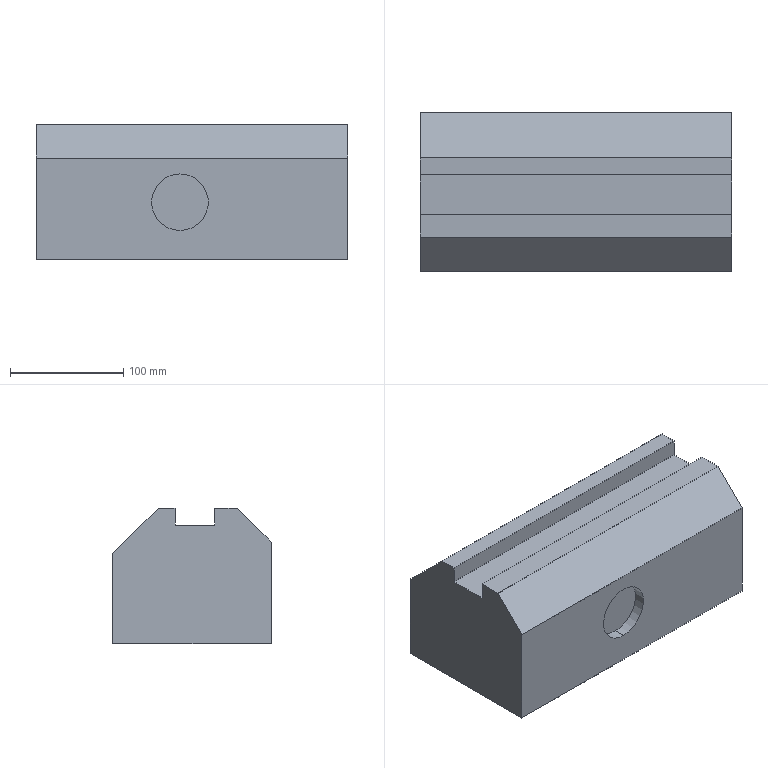CAM job | Mastercam | mm | 6 operations | part box 275 x 140 x 120
1. Pocket (Standard) | 1 - 10 平铣刀
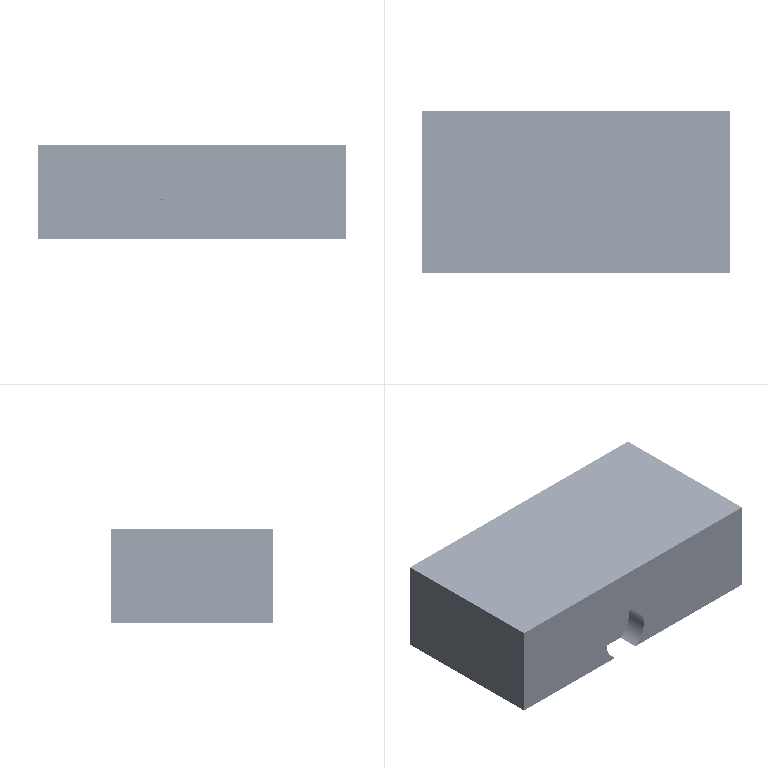2. Facing | 1 - 10 平铣刀
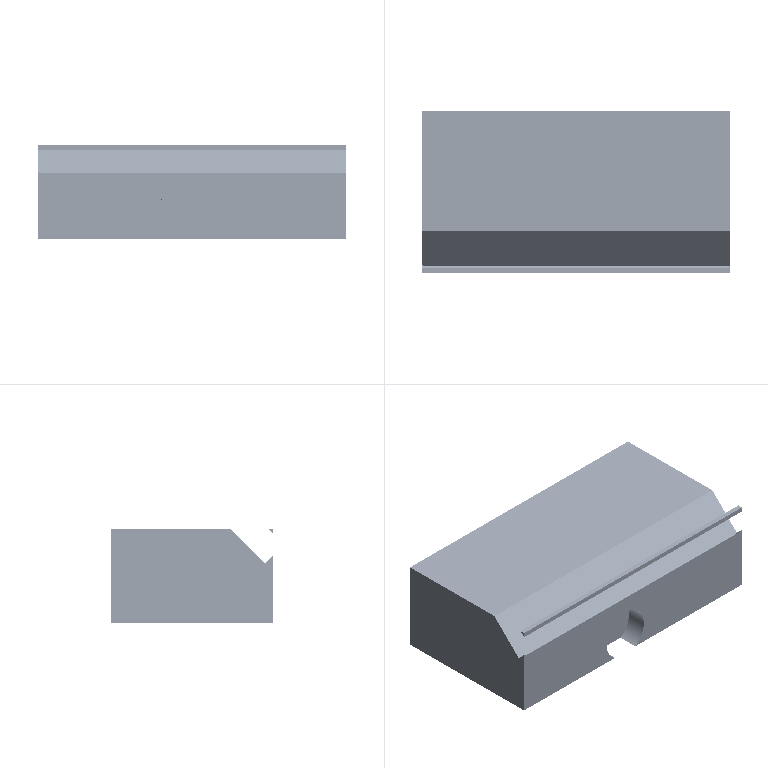3. 2D High Speed (2D Blend Mill) | 1 - 10 平铣刀
4. 2D High Speed (2D Blend Mill) | 1 - 10 平铣刀
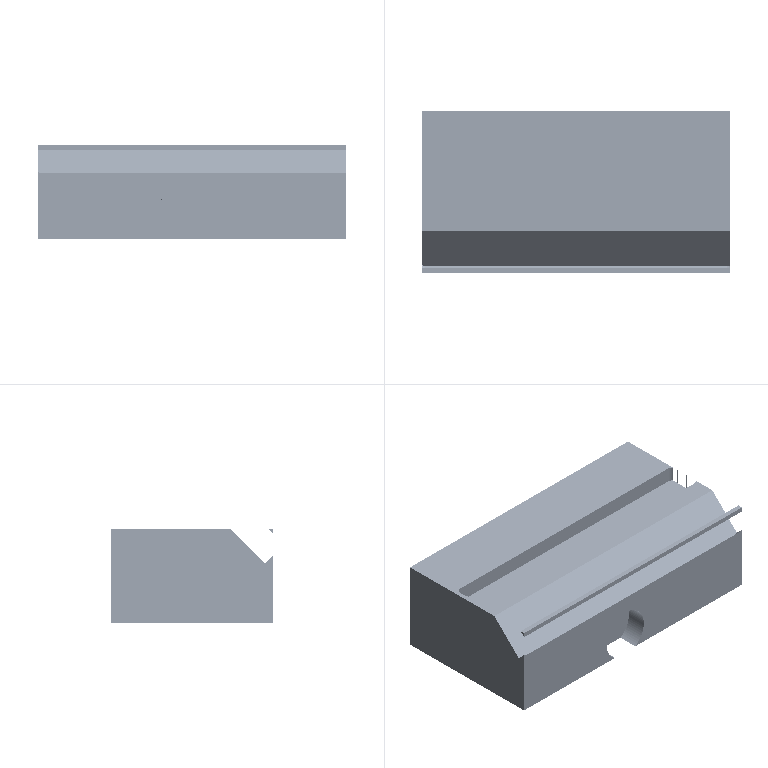5. Facing | 1 - 10 平铣刀
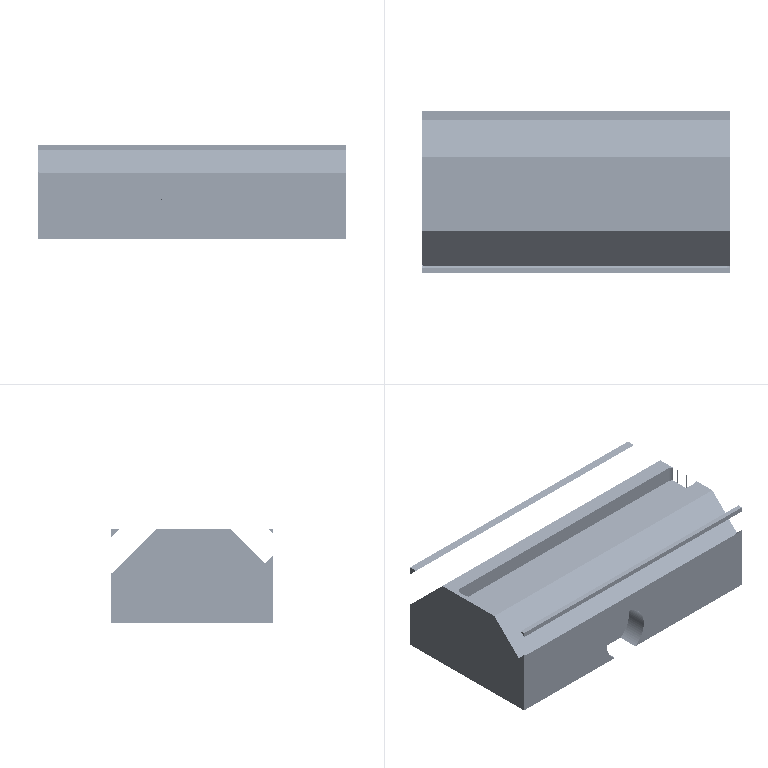6. Pocket (Standard) | 1 - 10 平铣刀